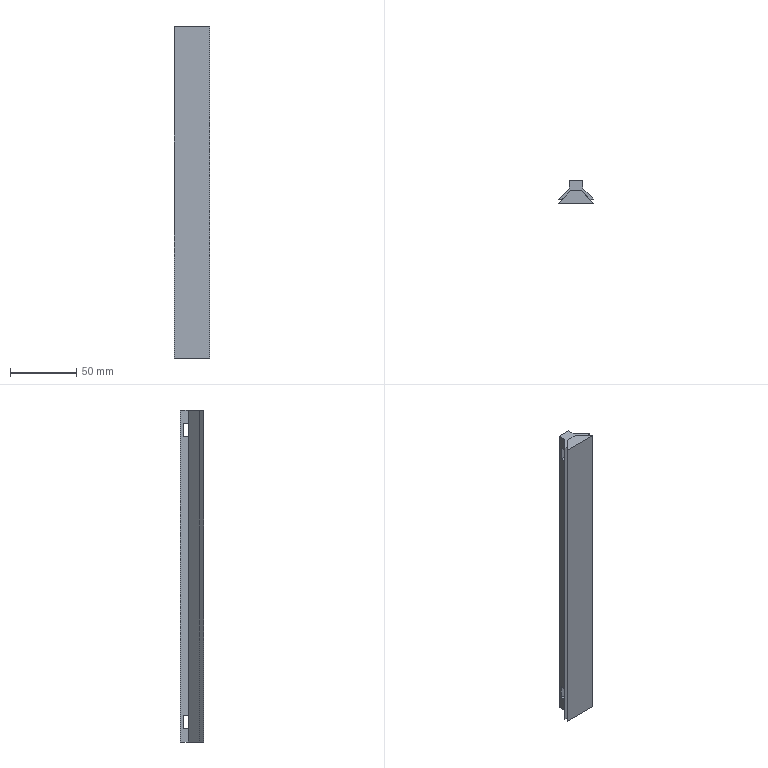Component | SolidWorks | Scraper-1 | 2 solids | 26 faces | box 26.97 x 17.45 x 250 mm | volume 70404 mm3 | plane 26
build123d program:
from build123d import *

# Parameters (mm, degrees)
BOSS_EXTRUDE1_DEPTH = 125
SKETCH3_W           = 250
SKETCH3_H           = 10
BOSS_EXTRUDE2_DEPTH = 6
SKETCH4_W           = 10
SKETCH4_H           = 4
CUT_EXTRUDE1_DEPTH  = 10
BOSS_EXTRUDE3_DEPTH = 250


with BuildPart() as part:
    # Sketch2 → Boss-Extrude1 (new, symmetric)
    with BuildSketch(Plane(origin=(0, 0, 0), x_dir=(0, 0, -1), z_dir=(1, 0, 0))):
        Polygon((-5, 0), (5, 0), (13.266, -8.266), (10.438, -8.266), (4.172, -2), (-4.172, -2), (-10.657, -8.485), (-13.485, -8.485), align=None)
    extrude(amount=BOSS_EXTRUDE1_DEPTH, both=True)

    # Sketch3 → Boss-Extrude2 (add)
    with BuildSketch(Plane(origin=(0, 0, 0), x_dir=(1, 0, 0), z_dir=(0, 1, 0))):
        Rectangle(SKETCH3_W, SKETCH3_H)
    extrude(amount=BOSS_EXTRUDE2_DEPTH)

    # Sketch4 → Cut-Extrude1 (cut)
    with BuildSketch(Plane.XY.offset(5)):
        with Locations((-110, 2)):
            Rectangle(SKETCH4_W, SKETCH4_H)
        with Locations((110, 2)):
            Rectangle(SKETCH4_W, SKETCH4_H)
    extrude(amount=-CUT_EXTRUDE1_DEPTH, mode=Mode.SUBTRACT)


with BuildPart() as body_2:
    # Sketch5 → Boss-Extrude3 (new body)
    with BuildSketch(Plane.ZY.offset(125)):
        Polygon((-4.13, -2.1), (-13.484, -11.453), (13.484, -11.453), (4.13, -2.1), align=None)
    extrude(amount=-BOSS_EXTRUDE3_DEPTH)


solid = Compound([part.part, body_2.part])

# Placed as in the assembly
solid = solid.moved(Location((440.482, -390.1, -8.037), (0, -90, 0)))
STEP:
#1=COLOUR_RGB('',0.7922,0.8196,0.9333);
#2=FILL_AREA_STYLE_COLOUR('',#1);
#3=FILL_AREA_STYLE('',(#2));
#4=SURFACE_STYLE_FILL_AREA(#3);
#5=SURFACE_SIDE_STYLE('',(#4));
#6=SURFACE_STYLE_USAGE(.BOTH.,#5);
#7=PRESENTATION_STYLE_ASSIGNMENT((#6));
#8=CARTESIAN_POINT('',(17.145,-15.358,-5.238));
#9=VERTEX_POINT('',#8);
#10=CARTESIAN_POINT('',(16.811,-15.692,-5.238));
#11=VERTEX_POINT('',#10);
#12=CARTESIAN_POINT('',(17.145,-15.358,-5.238));
#13=DIRECTION('',(-0.7071,-0.7071,-0.));
#14=VECTOR('',#13,39.37);
#15=LINE('',#12,#14);
#16=EDGE_CURVE('',#9,#11,#15,.T.);
#17=ORIENTED_EDGE('',*,*,#16,.T.);
#18=CARTESIAN_POINT('',(16.811,-15.692,4.605));
#19=VERTEX_POINT('',#18);
#20=CARTESIAN_POINT('',(16.811,-15.692,4.605));
#21=DIRECTION('',(0.,-0.,-1.));
#22=VECTOR('',#21,39.37);
#23=LINE('',#20,#22);
#24=EDGE_CURVE('',#19,#11,#23,.T.);
#25=ORIENTED_EDGE('',*,*,#24,.F.);
#26=CARTESIAN_POINT('',(17.145,-15.358,4.605));
#27=VERTEX_POINT('',#26);
#28=CARTESIAN_POINT('',(17.145,-15.358,4.605));
#29=DIRECTION('',(-0.7071,-0.7071,-0.));
#30=VECTOR('',#29,39.37);
#31=LINE('',#28,#30);
#32=EDGE_CURVE('',#27,#19,#31,.T.);
#33=ORIENTED_EDGE('',*,*,#32,.F.);
#34=CARTESIAN_POINT('',(17.145,-15.358,4.211));
#35=VERTEX_POINT('',#34);
#36=CARTESIAN_POINT('',(17.145,-15.358,4.605));
#37=DIRECTION('',(0.,-0.,-1.));
#38=VECTOR('',#37,39.37);
#39=LINE('',#36,#38);
#40=EDGE_CURVE('',#27,#35,#39,.T.);
#41=ORIENTED_EDGE('',*,*,#40,.T.);
#42=CARTESIAN_POINT('',(17.145,-15.358,3.817));
#43=VERTEX_POINT('',#42);
#44=CARTESIAN_POINT('',(17.145,-15.358,4.211));
#45=DIRECTION('',(-0.,0.,1.));
#46=VECTOR('',#45,39.37);
#47=LINE('',#44,#46);
#48=EDGE_CURVE('',#43,#35,#47,.T.);
#49=ORIENTED_EDGE('',*,*,#48,.F.);
#50=CARTESIAN_POINT('',(17.145,-15.358,-4.45));
#51=VERTEX_POINT('',#50);
#52=CARTESIAN_POINT('',(17.145,-15.358,4.605));
#53=DIRECTION('',(0.,-0.,-1.));
#54=VECTOR('',#53,39.37);
#55=LINE('',#52,#54);
#56=EDGE_CURVE('',#43,#51,#55,.T.);
#57=ORIENTED_EDGE('',*,*,#56,.T.);
#58=CARTESIAN_POINT('',(17.145,-15.358,-4.844));
#59=VERTEX_POINT('',#58);
#60=CARTESIAN_POINT('',(17.145,-15.358,-4.844));
#61=DIRECTION('',(-0.,0.,1.));
#62=VECTOR('',#61,39.37);
#63=LINE('',#60,#62);
#64=EDGE_CURVE('',#59,#51,#63,.T.);
#65=ORIENTED_EDGE('',*,*,#64,.F.);
#66=CARTESIAN_POINT('',(17.145,-15.358,4.605));
#67=DIRECTION('',(0.,-0.,-1.));
#68=VECTOR('',#67,39.37);
#69=LINE('',#66,#68);
#70=EDGE_CURVE('',#59,#9,#69,.T.);
#71=ORIENTED_EDGE('',*,*,#70,.T.);
#72=EDGE_LOOP('',(#17,#25,#33,#41,#49,#57,#65,#71));
#73=FACE_OUTER_BOUND('',#72,.T.);
#74=CARTESIAN_POINT('',(17.145,-15.358,4.605));
#75=DIRECTION('',(0.7071,-0.7071,0.));
#76=DIRECTION('',(0.7071,0.7071,0.));
#77=AXIS2_PLACEMENT_3D('',#74,#75,#76);
#78=PLANE('',#77);
#79=ADVANCED_FACE('',(#73),#78,.F.);
#80=CARTESIAN_POINT('',(16.922,-15.692,-5.238));
#81=VERTEX_POINT('',#80);
#82=CARTESIAN_POINT('',(16.922,-15.692,-5.238));
#83=DIRECTION('',(1.,0.,0.));
#84=VECTOR('',#83,39.37);
#85=LINE('',#82,#84);
#86=EDGE_CURVE('',#11,#81,#85,.T.);
#87=ORIENTED_EDGE('',*,*,#86,.T.);
#88=CARTESIAN_POINT('',(16.922,-15.692,4.605));
#89=VERTEX_POINT('',#88);
#90=CARTESIAN_POINT('',(16.922,-15.692,4.605));
#91=DIRECTION('',(0.,-0.,-1.));
#92=VECTOR('',#91,39.37);
#93=LINE('',#90,#92);
#94=EDGE_CURVE('',#89,#81,#93,.T.);
#95=ORIENTED_EDGE('',*,*,#94,.F.);
#96=CARTESIAN_POINT('',(16.922,-15.692,4.605));
#97=DIRECTION('',(1.,0.,0.));
#98=VECTOR('',#97,39.37);
#99=LINE('',#96,#98);
#100=EDGE_CURVE('',#19,#89,#99,.T.);
#101=ORIENTED_EDGE('',*,*,#100,.F.);
#102=ORIENTED_EDGE('',*,*,#24,.T.);
#103=EDGE_LOOP('',(#87,#95,#101,#102));
#104=FACE_OUTER_BOUND('',#103,.T.);
#105=CARTESIAN_POINT('',(16.922,-15.692,4.605));
#106=DIRECTION('',(-0.,1.,-0.));
#107=DIRECTION('',(-1.,-0.,-0.));
#108=AXIS2_PLACEMENT_3D('',#105,#106,#107);
#109=PLANE('',#108);
#110=ADVANCED_FACE('',(#104),#109,.F.);
#111=CARTESIAN_POINT('',(17.178,-15.437,-5.238));
#112=VERTEX_POINT('',#111);
#113=CARTESIAN_POINT('',(17.178,-15.437,-5.238));
#114=DIRECTION('',(0.7071,0.7071,0.));
#115=VECTOR('',#114,39.37);
#116=LINE('',#113,#115);
#117=EDGE_CURVE('',#81,#112,#116,.T.);
#118=ORIENTED_EDGE('',*,*,#117,.T.);
#119=CARTESIAN_POINT('',(17.178,-15.437,4.605));
#120=VERTEX_POINT('',#119);
#121=CARTESIAN_POINT('',(17.178,-15.437,4.605));
#122=DIRECTION('',(0.,-0.,-1.));
#123=VECTOR('',#122,39.37);
#124=LINE('',#121,#123);
#125=EDGE_CURVE('',#120,#112,#124,.T.);
#126=ORIENTED_EDGE('',*,*,#125,.F.);
#127=CARTESIAN_POINT('',(17.178,-15.437,4.605));
#128=DIRECTION('',(0.7071,0.7071,0.));
#129=VECTOR('',#128,39.37);
#130=LINE('',#127,#129);
#131=EDGE_CURVE('',#89,#120,#130,.T.);
#132=ORIENTED_EDGE('',*,*,#131,.F.);
#133=ORIENTED_EDGE('',*,*,#94,.T.);
#134=EDGE_LOOP('',(#118,#126,#132,#133));
#135=FACE_OUTER_BOUND('',#134,.T.);
#136=CARTESIAN_POINT('',(17.178,-15.437,4.605));
#137=DIRECTION('',(-0.7071,0.7071,-0.));
#138=DIRECTION('',(-0.7071,-0.7071,-0.));
#139=AXIS2_PLACEMENT_3D('',#136,#137,#138);
#140=PLANE('',#139);
#141=ADVANCED_FACE('',(#135),#140,.F.);
#142=CARTESIAN_POINT('',(17.506,-15.437,-5.238));
#143=VERTEX_POINT('',#142);
#144=CARTESIAN_POINT('',(17.178,-15.437,-5.238));
#145=DIRECTION('',(1.,0.,0.));
#146=VECTOR('',#145,39.37);
#147=LINE('',#144,#146);
#148=EDGE_CURVE('',#112,#143,#147,.T.);
#149=ORIENTED_EDGE('',*,*,#148,.T.);
#150=CARTESIAN_POINT('',(17.506,-15.437,4.605));
#151=VERTEX_POINT('',#150);
#152=CARTESIAN_POINT('',(17.506,-15.437,4.605));
#153=DIRECTION('',(0.,-0.,-1.));
#154=VECTOR('',#153,39.37);
#155=LINE('',#152,#154);
#156=EDGE_CURVE('',#151,#143,#155,.T.);
#157=ORIENTED_EDGE('',*,*,#156,.F.);
#158=CARTESIAN_POINT('',(17.178,-15.437,4.605));
#159=DIRECTION('',(1.,0.,0.));
#160=VECTOR('',#159,39.37);
#161=LINE('',#158,#160);
#162=EDGE_CURVE('',#120,#151,#161,.T.);
#163=ORIENTED_EDGE('',*,*,#162,.F.);
#164=ORIENTED_EDGE('',*,*,#125,.T.);
#165=EDGE_LOOP('',(#149,#157,#163,#164));
#166=FACE_OUTER_BOUND('',#165,.T.);
#167=CARTESIAN_POINT('',(17.178,-15.437,4.605));
#168=DIRECTION('',(-0.,1.,-0.));
#169=DIRECTION('',(-1.,-0.,-0.));
#170=AXIS2_PLACEMENT_3D('',#167,#168,#169);
#171=PLANE('',#170);
#172=ADVANCED_FACE('',(#166),#171,.F.);
#173=CARTESIAN_POINT('',(17.753,-15.684,-5.238));
#174=VERTEX_POINT('',#173);
#175=CARTESIAN_POINT('',(17.506,-15.437,-5.238));
#176=DIRECTION('',(0.7071,-0.7071,0.));
#177=VECTOR('',#176,39.37);
#178=LINE('',#175,#177);
#179=EDGE_CURVE('',#143,#174,#178,.T.);
#180=ORIENTED_EDGE('',*,*,#179,.T.);
#181=CARTESIAN_POINT('',(17.753,-15.684,4.605));
#182=VERTEX_POINT('',#181);
#183=CARTESIAN_POINT('',(17.753,-15.684,4.605));
#184=DIRECTION('',(0.,-0.,-1.));
#185=VECTOR('',#184,39.37);
#186=LINE('',#183,#185);
#187=EDGE_CURVE('',#182,#174,#186,.T.);
#188=ORIENTED_EDGE('',*,*,#187,.F.);
#189=CARTESIAN_POINT('',(17.506,-15.437,4.605));
#190=DIRECTION('',(0.7071,-0.7071,0.));
#191=VECTOR('',#190,39.37);
#192=LINE('',#189,#191);
#193=EDGE_CURVE('',#151,#182,#192,.T.);
#194=ORIENTED_EDGE('',*,*,#193,.F.);
#195=ORIENTED_EDGE('',*,*,#156,.T.);
#196=EDGE_LOOP('',(#180,#188,#194,#195));
#197=FACE_OUTER_BOUND('',#196,.T.);
#198=CARTESIAN_POINT('',(17.506,-15.437,4.605));
#199=DIRECTION('',(0.7071,0.7071,0.));
#200=DIRECTION('',(-0.7071,0.7071,-0.));
#201=AXIS2_PLACEMENT_3D('',#198,#199,#200);
#202=PLANE('',#201);
#203=ADVANCED_FACE('',(#197),#202,.F.);
#204=CARTESIAN_POINT('',(17.864,-15.684,-5.238));
#205=VERTEX_POINT('',#204);
#206=CARTESIAN_POINT('',(17.753,-15.684,-5.238));
#207=DIRECTION('',(1.,0.,0.));
#208=VECTOR('',#207,39.37);
#209=LINE('',#206,#208);
#210=EDGE_CURVE('',#174,#205,#209,.T.);
#211=ORIENTED_EDGE('',*,*,#210,.T.);
#212=CARTESIAN_POINT('',(17.864,-15.684,4.605));
#213=VERTEX_POINT('',#212);
#214=CARTESIAN_POINT('',(17.864,-15.684,4.605));
#215=DIRECTION('',(0.,-0.,-1.));
#216=VECTOR('',#215,39.37);
#217=LINE('',#214,#216);
#218=EDGE_CURVE('',#213,#205,#217,.T.);
#219=ORIENTED_EDGE('',*,*,#218,.F.);
#220=CARTESIAN_POINT('',(17.753,-15.684,4.605));
#221=DIRECTION('',(1.,0.,0.));
#222=VECTOR('',#221,39.37);
#223=LINE('',#220,#222);
#224=EDGE_CURVE('',#182,#213,#223,.T.);
#225=ORIENTED_EDGE('',*,*,#224,.F.);
#226=ORIENTED_EDGE('',*,*,#187,.T.);
#227=EDGE_LOOP('',(#211,#219,#225,#226));
#228=FACE_OUTER_BOUND('',#227,.T.);
#229=CARTESIAN_POINT('',(17.753,-15.684,4.605));
#230=DIRECTION('',(-0.,1.,-0.));
#231=DIRECTION('',(-1.,-0.,-0.));
#232=AXIS2_PLACEMENT_3D('',#229,#230,#231);
#233=PLANE('',#232);
#234=ADVANCED_FACE('',(#228),#233,.F.);
#235=CARTESIAN_POINT('',(17.539,-15.358,-5.238));
#236=VERTEX_POINT('',#235);
#237=CARTESIAN_POINT('',(17.539,-15.358,-5.238));
#238=DIRECTION('',(-0.7071,0.7071,-0.));
#239=VECTOR('',#238,39.37);
#240=LINE('',#237,#239);
#241=EDGE_CURVE('',#205,#236,#240,.T.);
#242=ORIENTED_EDGE('',*,*,#241,.T.);
#243=CARTESIAN_POINT('',(17.539,-15.358,-4.844));
#244=VERTEX_POINT('',#243);
#245=CARTESIAN_POINT('',(17.539,-15.358,4.605));
#246=DIRECTION('',(0.,-0.,-1.));
#247=VECTOR('',#246,39.37);
#248=LINE('',#245,#247);
#249=EDGE_CURVE('',#244,#236,#248,.T.);
#250=ORIENTED_EDGE('',*,*,#249,.F.);
#251=CARTESIAN_POINT('',(17.539,-15.358,-4.45));
#252=VERTEX_POINT('',#251);
#253=CARTESIAN_POINT('',(17.539,-15.358,-4.844));
#254=DIRECTION('',(-0.,0.,1.));
#255=VECTOR('',#254,39.37);
#256=LINE('',#253,#255);
#257=EDGE_CURVE('',#244,#252,#256,.T.);
#258=ORIENTED_EDGE('',*,*,#257,.T.);
#259=CARTESIAN_POINT('',(17.539,-15.358,3.817));
#260=VERTEX_POINT('',#259);
#261=CARTESIAN_POINT('',(17.539,-15.358,4.605));
#262=DIRECTION('',(0.,-0.,-1.));
#263=VECTOR('',#262,39.37);
#264=LINE('',#261,#263);
#265=EDGE_CURVE('',#260,#252,#264,.T.);
#266=ORIENTED_EDGE('',*,*,#265,.F.);
#267=CARTESIAN_POINT('',(17.539,-15.358,4.211));
#268=VERTEX_POINT('',#267);
#269=CARTESIAN_POINT('',(17.539,-15.358,4.211));
#270=DIRECTION('',(-0.,0.,1.));
#271=VECTOR('',#270,39.37);
#272=LINE('',#269,#271);
#273=EDGE_CURVE('',#260,#268,#272,.T.);
#274=ORIENTED_EDGE('',*,*,#273,.T.);
#275=CARTESIAN_POINT('',(17.539,-15.358,4.605));
#276=VERTEX_POINT('',#275);
#277=CARTESIAN_POINT('',(17.539,-15.358,4.605));
#278=DIRECTION('',(0.,-0.,-1.));
#279=VECTOR('',#278,39.37);
#280=LINE('',#277,#279);
#281=EDGE_CURVE('',#276,#268,#280,.T.);
#282=ORIENTED_EDGE('',*,*,#281,.F.);
#283=CARTESIAN_POINT('',(17.539,-15.358,4.605));
#284=DIRECTION('',(-0.7071,0.7071,-0.));
#285=VECTOR('',#284,39.37);
#286=LINE('',#283,#285);
#287=EDGE_CURVE('',#213,#276,#286,.T.);
#288=ORIENTED_EDGE('',*,*,#287,.F.);
#289=ORIENTED_EDGE('',*,*,#218,.T.);
#290=EDGE_LOOP('',(#242,#250,#258,#266,#274,#282,#288,#289));
#291=FACE_OUTER_BOUND('',#290,.T.);
#292=CARTESIAN_POINT('',(17.539,-15.358,4.605));
#293=DIRECTION('',(-0.7071,-0.7071,-0.));
#294=DIRECTION('',(0.7071,-0.7071,0.));
#295=AXIS2_PLACEMENT_3D('',#292,#293,#294);
#296=PLANE('',#295);
#297=ADVANCED_FACE('',(#291),#296,.F.);
#298=ORIENTED_EDGE('',*,*,#32,.T.);
#299=ORIENTED_EDGE('',*,*,#100,.T.);
#300=ORIENTED_EDGE('',*,*,#131,.T.);
#301=ORIENTED_EDGE('',*,*,#162,.T.);
#302=ORIENTED_EDGE('',*,*,#193,.T.);
#303=ORIENTED_EDGE('',*,*,#224,.T.);
#304=ORIENTED_EDGE('',*,*,#287,.T.);
#305=CARTESIAN_POINT('',(17.539,-15.122,4.605));
#306=VERTEX_POINT('',#305);
#307=CARTESIAN_POINT('',(17.539,-15.122,4.605));
#308=DIRECTION('',(0.,-1.,0.));
#309=VECTOR('',#308,39.37);
#310=LINE('',#307,#309);
#311=EDGE_CURVE('',#306,#276,#310,.T.);
#312=ORIENTED_EDGE('',*,*,#311,.F.);
#313=CARTESIAN_POINT('',(17.145,-15.122,4.605));
#314=VERTEX_POINT('',#313);
#315=CARTESIAN_POINT('',(17.145,-15.122,4.605));
#316=DIRECTION('',(1.,0.,0.));
#317=VECTOR('',#316,39.37);
#318=LINE('',#315,#317);
#319=EDGE_CURVE('',#314,#306,#318,.T.);
#320=ORIENTED_EDGE('',*,*,#319,.F.);
#321=CARTESIAN_POINT('',(17.145,-15.122,4.605));
#322=DIRECTION('',(0.,-1.,0.));
#323=VECTOR('',#322,39.37);
#324=LINE('',#321,#323);
#325=EDGE_CURVE('',#314,#27,#324,.T.);
#326=ORIENTED_EDGE('',*,*,#325,.T.);
#327=EDGE_LOOP('',(#298,#299,#300,#301,#302,#303,#304,#312,#320,#326));
#328=FACE_OUTER_BOUND('',#327,.T.);
#329=CARTESIAN_POINT('',(17.342,-15.358,4.605));
#330=DIRECTION('',(-0.,0.,1.));
#331=DIRECTION('',(1.,0.,0.));
#332=AXIS2_PLACEMENT_3D('',#329,#330,#331);
#333=PLANE('',#332);
#334=ADVANCED_FACE('',(#328),#333,.T.);
#335=ORIENTED_EDGE('',*,*,#16,.F.);
#336=CARTESIAN_POINT('',(17.145,-15.122,-5.238));
#337=VERTEX_POINT('',#336);
#338=CARTESIAN_POINT('',(17.145,-15.122,-5.238));
#339=DIRECTION('',(0.,-1.,0.));
#340=VECTOR('',#339,39.37);
#341=LINE('',#338,#340);
#342=EDGE_CURVE('',#337,#9,#341,.T.);
#343=ORIENTED_EDGE('',*,*,#342,.F.);
#344=CARTESIAN_POINT('',(17.539,-15.122,-5.238));
#345=VERTEX_POINT('',#344);
#346=CARTESIAN_POINT('',(17.145,-15.122,-5.238));
#347=DIRECTION('',(-1.,-0.,-0.));
#348=VECTOR('',#347,39.37);
#349=LINE('',#346,#348);
#350=EDGE_CURVE('',#345,#337,#349,.T.);
#351=ORIENTED_EDGE('',*,*,#350,.F.);
#352=CARTESIAN_POINT('',(17.539,-15.122,-5.238));
#353=DIRECTION('',(0.,-1.,0.));
#354=VECTOR('',#353,39.37);
#355=LINE('',#352,#354);
#356=EDGE_CURVE('',#345,#236,#355,.T.);
#357=ORIENTED_EDGE('',*,*,#356,.T.);
#358=ORIENTED_EDGE('',*,*,#241,.F.);
#359=ORIENTED_EDGE('',*,*,#210,.F.);
#360=ORIENTED_EDGE('',*,*,#179,.F.);
#361=ORIENTED_EDGE('',*,*,#148,.F.);
#362=ORIENTED_EDGE('',*,*,#117,.F.);
#363=ORIENTED_EDGE('',*,*,#86,.F.);
#364=EDGE_LOOP('',(#335,#343,#351,#357,#358,#359,#360,#361,#362,#363));
#365=FACE_OUTER_BOUND('',#364,.T.);
#366=CARTESIAN_POINT('',(17.342,-15.358,-5.238));
#367=DIRECTION('',(-0.,0.,1.));
#368=DIRECTION('',(1.,0.,0.));
#369=AXIS2_PLACEMENT_3D('',#366,#367,#368);
#370=PLANE('',#369);
#371=ADVANCED_FACE('',(#365),#370,.F.);
#372=ORIENTED_EDGE('',*,*,#281,.T.);
#373=CARTESIAN_POINT('',(17.539,-15.201,4.211));
#374=VERTEX_POINT('',#373);
#375=CARTESIAN_POINT('',(17.539,-15.201,4.211));
#376=DIRECTION('',(-0.,1.,-0.));
#377=VECTOR('',#376,39.37);
#378=LINE('',#375,#377);
#379=EDGE_CURVE('',#268,#374,#378,.T.);
#380=ORIENTED_EDGE('',*,*,#379,.T.);
#381=CARTESIAN_POINT('',(17.539,-15.201,3.817));
#382=VERTEX_POINT('',#381);
#383=CARTESIAN_POINT('',(17.539,-15.201,3.817));
#384=DIRECTION('',(0.,-0.,-1.));
#385=VECTOR('',#384,39.37);
#386=LINE('',#383,#385);
#387=EDGE_CURVE('',#374,#382,#386,.T.);
#388=ORIENTED_EDGE('',*,*,#387,.T.);
#389=CARTESIAN_POINT('',(17.539,-15.358,3.817));
#390=DIRECTION('',(0.,-1.,0.));
#391=VECTOR('',#390,39.37);
#392=LINE('',#389,#391);
#393=EDGE_CURVE('',#382,#260,#392,.T.);
#394=ORIENTED_EDGE('',*,*,#393,.T.);
#395=ORIENTED_EDGE('',*,*,#265,.T.);
#396=CARTESIAN_POINT('',(17.539,-15.201,-4.45));
#397=VERTEX_POINT('',#396);
#398=CARTESIAN_POINT('',(17.539,-15.358,-4.45));
#399=DIRECTION('',(-0.,1.,-0.));
#400=VECTOR('',#399,39.37);
#401=LINE('',#398,#400);
#402=EDGE_CURVE('',#252,#397,#401,.T.);
#403=ORIENTED_EDGE('',*,*,#402,.T.);
#404=CARTESIAN_POINT('',(17.539,-15.201,-4.844));
#405=VERTEX_POINT('',#404);
#406=CARTESIAN_POINT('',(17.539,-15.201,-4.45));
#407=DIRECTION('',(0.,-0.,-1.));
#408=VECTOR('',#407,39.37);
#409=LINE('',#406,#408);
#410=EDGE_CURVE('',#397,#405,#409,.T.);
#411=ORIENTED_EDGE('',*,*,#410,.T.);
#412=CARTESIAN_POINT('',(17.539,-15.201,-4.844));
#413=DIRECTION('',(0.,-1.,0.));
#414=VECTOR('',#413,39.37);
#415=LINE('',#412,#414);
#416=EDGE_CURVE('',#405,#244,#415,.T.);
#417=ORIENTED_EDGE('',*,*,#416,.T.);
#418=ORIENTED_EDGE('',*,*,#249,.T.);
#419=ORIENTED_EDGE('',*,*,#356,.F.);
#420=CARTESIAN_POINT('',(17.539,-15.122,-5.238));
#421=DIRECTION('',(0.,-0.,-1.));
#422=VECTOR('',#421,39.37);
#423=LINE('',#420,#422);
#424=EDGE_CURVE('',#306,#345,#423,.T.);
#425=ORIENTED_EDGE('',*,*,#424,.F.);
#426=ORIENTED_EDGE('',*,*,#311,.T.);
#427=EDGE_LOOP('',(#372,#380,#388,#394,#395,#403,#411,#417,#418,#419,#425,#426));
#428=FACE_OUTER_BOUND('',#427,.T.);
#429=CARTESIAN_POINT('',(17.539,-15.122,-5.238));
#430=DIRECTION('',(-1.,-0.,-0.));
#431=DIRECTION('',(0.,-1.,0.));
#432=AXIS2_PLACEMENT_3D('',#429,#430,#431);
#433=PLANE('',#432);
#434=ADVANCED_FACE('',(#428),#433,.F.);
#435=CARTESIAN_POINT('',(17.145,-15.201,4.211));
#436=VERTEX_POINT('',#435);
#437=CARTESIAN_POINT('',(17.145,-15.201,3.817));
#438=VERTEX_POINT('',#437);
#439=CARTESIAN_POINT('',(17.145,-15.201,3.817));
#440=DIRECTION('',(0.,-0.,-1.));
#441=VECTOR('',#440,39.37);
#442=LINE('',#439,#441);
#443=EDGE_CURVE('',#436,#438,#442,.T.);
#444=ORIENTED_EDGE('',*,*,#443,.F.);
#445=CARTESIAN_POINT('',(17.145,-15.201,4.211));
#446=DIRECTION('',(-0.,1.,-0.));
#447=VECTOR('',#446,39.37);
#448=LINE('',#445,#447);
#449=EDGE_CURVE('',#35,#436,#448,.T.);
#450=ORIENTED_EDGE('',*,*,#449,.F.);
#451=ORIENTED_EDGE('',*,*,#40,.F.);
#452=ORIENTED_EDGE('',*,*,#325,.F.);
#453=CARTESIAN_POINT('',(17.145,-15.122,-5.238));
#454=DIRECTION('',(-0.,0.,1.));
#455=VECTOR('',#454,39.37);
#456=LINE('',#453,#455);
#457=EDGE_CURVE('',#337,#314,#456,.T.);
#458=ORIENTED_EDGE('',*,*,#457,.F.);
#459=ORIENTED_EDGE('',*,*,#342,.T.);
#460=ORIENTED_EDGE('',*,*,#70,.F.);
#461=CARTESIAN_POINT('',(17.145,-15.201,-4.844));
#462=VERTEX_POINT('',#461);
#463=CARTESIAN_POINT('',(17.145,-15.201,-4.844));
#464=DIRECTION('',(0.,-1.,0.));
#465=VECTOR('',#464,39.37);
#466=LINE('',#463,#465);
#467=EDGE_CURVE('',#462,#59,#466,.T.);
#468=ORIENTED_EDGE('',*,*,#467,.F.);
#469=CARTESIAN_POINT('',(17.145,-15.201,-4.45));
#470=VERTEX_POINT('',#469);
#471=CARTESIAN_POINT('',(17.145,-15.201,-4.45));
#472=DIRECTION('',(0.,-0.,-1.));
#473=VECTOR('',#472,39.37);
#474=LINE('',#471,#473);
#475=EDGE_CURVE('',#470,#462,#474,.T.);
#476=ORIENTED_EDGE('',*,*,#475,.F.);
#477=CARTESIAN_POINT('',(17.145,-15.358,-4.45));
#478=DIRECTION('',(-0.,1.,-0.));
#479=VECTOR('',#478,39.37);
#480=LINE('',#477,#479);
#481=EDGE_CURVE('',#51,#470,#480,.T.);
#482=ORIENTED_EDGE('',*,*,#481,.F.);
#483=ORIENTED_EDGE('',*,*,#56,.F.);
#484=CARTESIAN_POINT('',(17.145,-15.358,3.817));
#485=DIRECTION('',(0.,-1.,0.));
#486=VECTOR('',#485,39.37);
#487=LINE('',#484,#486);
#488=EDGE_CURVE('',#438,#43,#487,.T.);
#489=ORIENTED_EDGE('',*,*,#488,.F.);
#490=EDGE_LOOP('',(#444,#450,#451,#452,#458,#459,#460,#468,#476,#482,#483,#489));
#491=FACE_OUTER_BOUND('',#490,.T.);
#492=CARTESIAN_POINT('',(17.145,-15.122,-5.238));
#493=DIRECTION('',(1.,0.,0.));
#494=DIRECTION('',(-0.,1.,-0.));
#495=AXIS2_PLACEMENT_3D('',#492,#493,#494);
#496=PLANE('',#495);
#497=ADVANCED_FACE('',(#491),#496,.F.);
#498=ORIENTED_EDGE('',*,*,#319,.T.);
#499=ORIENTED_EDGE('',*,*,#424,.T.);
#500=ORIENTED_EDGE('',*,*,#350,.T.);
#501=ORIENTED_EDGE('',*,*,#457,.T.);
#502=EDGE_LOOP('',(#498,#499,#500,#501));
#503=FACE_OUTER_BOUND('',#502,.T.);
#504=CARTESIAN_POINT('',(17.342,-15.122,-0.3164));
#505=DIRECTION('',(0.,-1.,0.));
#506=DIRECTION('',(1.,0.,0.));
#507=AXIS2_PLACEMENT_3D('',#504,#505,#506);
#508=PLANE('',#507);
#509=ADVANCED_FACE('',(#503),#508,.F.);
#510=ORIENTED_EDGE('',*,*,#64,.T.);
#511=CARTESIAN_POINT('',(17.539,-15.358,-4.45));
#512=DIRECTION('',(-1.,-0.,-0.));
#513=VECTOR('',#512,39.37);
#514=LINE('',#511,#513);
#515=EDGE_CURVE('',#252,#51,#514,.T.);
#516=ORIENTED_EDGE('',*,*,#515,.F.);
#517=ORIENTED_EDGE('',*,*,#257,.F.);
#518=CARTESIAN_POINT('',(17.539,-15.358,-4.844));
#519=DIRECTION('',(-1.,-0.,-0.));
#520=VECTOR('',#519,39.37);
#521=LINE('',#518,#520);
#522=EDGE_CURVE('',#244,#59,#521,.T.);
#523=ORIENTED_EDGE('',*,*,#522,.T.);
#524=EDGE_LOOP('',(#510,#516,#517,#523));
#525=FACE_OUTER_BOUND('',#524,.T.);
#526=CARTESIAN_POINT('',(17.539,-15.358,-4.844));
#527=DIRECTION('',(0.,-1.,0.));
#528=DIRECTION('',(-0.,0.,1.));
#529=AXIS2_PLACEMENT_3D('',#526,#527,#528);
#530=PLANE('',#529);
#531=ADVANCED_FACE('',(#525),#530,.F.);
#532=ORIENTED_EDGE('',*,*,#467,.T.);
#533=ORIENTED_EDGE('',*,*,#522,.F.);
#534=ORIENTED_EDGE('',*,*,#416,.F.);
#535=CARTESIAN_POINT('',(17.539,-15.201,-4.844));
#536=DIRECTION('',(-1.,-0.,-0.));
#537=VECTOR('',#536,39.37);
#538=LINE('',#535,#537);
#539=EDGE_CURVE('',#405,#462,#538,.T.);
#540=ORIENTED_EDGE('',*,*,#539,.T.);
#541=EDGE_LOOP('',(#532,#533,#534,#540));
#542=FACE_OUTER_BOUND('',#541,.T.);
#543=CARTESIAN_POINT('',(17.539,-15.201,-4.844));
#544=DIRECTION('',(0.,-0.,-1.));
#545=DIRECTION('',(-1.,-0.,-0.));
#546=AXIS2_PLACEMENT_3D('',#543,#544,#545);
#547=PLANE('',#546);
#548=ADVANCED_FACE('',(#542),#547,.F.);
#549=ORIENTED_EDGE('',*,*,#475,.T.);
#550=ORIENTED_EDGE('',*,*,#539,.F.);
#551=ORIENTED_EDGE('',*,*,#410,.F.);
#552=CARTESIAN_POINT('',(17.539,-15.201,-4.45));
#553=DIRECTION('',(-1.,-0.,-0.));
#554=VECTOR('',#553,39.37);
#555=LINE('',#552,#554);
#556=EDGE_CURVE('',#397,#470,#555,.T.);
#557=ORIENTED_EDGE('',*,*,#556,.T.);
#558=EDGE_LOOP('',(#549,#550,#551,#557));
#559=FACE_OUTER_BOUND('',#558,.T.);
#560=CARTESIAN_POINT('',(17.539,-15.201,-4.45));
#561=DIRECTION('',(-0.,1.,-0.));
#562=DIRECTION('',(-1.,-0.,-0.));
#563=AXIS2_PLACEMENT_3D('',#560,#561,#562);
#564=PLANE('',#563);
#565=ADVANCED_FACE('',(#559),#564,.F.);
#566=ORIENTED_EDGE('',*,*,#481,.T.);
#567=ORIENTED_EDGE('',*,*,#556,.F.);
#568=ORIENTED_EDGE('',*,*,#402,.F.);
#569=ORIENTED_EDGE('',*,*,#515,.T.);
#570=EDGE_LOOP('',(#566,#567,#568,#569));
#571=FACE_OUTER_BOUND('',#570,.T.);
#572=CARTESIAN_POINT('',(17.539,-15.358,-4.45));
#573=DIRECTION('',(-0.,0.,1.));
#574=DIRECTION('',(1.,0.,0.));
#575=AXIS2_PLACEMENT_3D('',#572,#573,#574);
#576=PLANE('',#575);
#577=ADVANCED_FACE('',(#571),#576,.F.);
#578=ORIENTED_EDGE('',*,*,#449,.T.);
#579=CARTESIAN_POINT('',(17.539,-15.201,4.211));
#580=DIRECTION('',(-1.,-0.,-0.));
#581=VECTOR('',#580,39.37);
#582=LINE('',#579,#581);
#583=EDGE_CURVE('',#374,#436,#582,.T.);
#584=ORIENTED_EDGE('',*,*,#583,.F.);
#585=ORIENTED_EDGE('',*,*,#379,.F.);
#586=CARTESIAN_POINT('',(17.539,-15.358,4.211));
#587=DIRECTION('',(-1.,-0.,-0.));
#588=VECTOR('',#587,39.37);
#589=LINE('',#586,#588);
#590=EDGE_CURVE('',#268,#35,#589,.T.);
#591=ORIENTED_EDGE('',*,*,#590,.T.);
#592=EDGE_LOOP('',(#578,#584,#585,#591));
#593=FACE_OUTER_BOUND('',#592,.T.);
#594=CARTESIAN_POINT('',(17.539,-15.201,4.211));
#595=DIRECTION('',(-0.,0.,1.));
#596=DIRECTION('',(1.,0.,0.));
#597=AXIS2_PLACEMENT_3D('',#594,#595,#596);
#598=PLANE('',#597);
#599=ADVANCED_FACE('',(#593),#598,.F.);
#600=ORIENTED_EDGE('',*,*,#48,.T.);
#601=ORIENTED_EDGE('',*,*,#590,.F.);
#602=ORIENTED_EDGE('',*,*,#273,.F.);
#603=CARTESIAN_POINT('',(17.539,-15.358,3.817));
#604=DIRECTION('',(-1.,-0.,-0.));
#605=VECTOR('',#604,39.37);
#606=LINE('',#603,#605);
#607=EDGE_CURVE('',#260,#43,#606,.T.);
#608=ORIENTED_EDGE('',*,*,#607,.T.);
#609=EDGE_LOOP('',(#600,#601,#602,#608));
#610=FACE_OUTER_BOUND('',#609,.T.);
#611=CARTESIAN_POINT('',(17.539,-15.358,4.211));
#612=DIRECTION('',(0.,-1.,0.));
#613=DIRECTION('',(-0.,0.,1.));
#614=AXIS2_PLACEMENT_3D('',#611,#612,#613);
#615=PLANE('',#614);
#616=ADVANCED_FACE('',(#610),#615,.F.);
#617=ORIENTED_EDGE('',*,*,#488,.T.);
#618=ORIENTED_EDGE('',*,*,#607,.F.);
#619=ORIENTED_EDGE('',*,*,#393,.F.);
#620=CARTESIAN_POINT('',(17.539,-15.201,3.817));
#621=DIRECTION('',(-1.,-0.,-0.));
#622=VECTOR('',#621,39.37);
#623=LINE('',#620,#622);
#624=EDGE_CURVE('',#382,#438,#623,.T.);
#625=ORIENTED_EDGE('',*,*,#624,.T.);
#626=EDGE_LOOP('',(#617,#618,#619,#625));
#627=FACE_OUTER_BOUND('',#626,.T.);
#628=CARTESIAN_POINT('',(17.539,-15.358,3.817));
#629=DIRECTION('',(0.,-0.,-1.));
#630=DIRECTION('',(-1.,-0.,-0.));
#631=AXIS2_PLACEMENT_3D('',#628,#629,#630);
#632=PLANE('',#631);
#633=ADVANCED_FACE('',(#627),#632,.F.);
#634=ORIENTED_EDGE('',*,*,#443,.T.);
#635=ORIENTED_EDGE('',*,*,#624,.F.);
#636=ORIENTED_EDGE('',*,*,#387,.F.);
#637=ORIENTED_EDGE('',*,*,#583,.T.);
#638=EDGE_LOOP('',(#634,#635,#636,#637));
#639=FACE_OUTER_BOUND('',#638,.T.);
#640=CARTESIAN_POINT('',(17.539,-15.201,3.817));
#641=DIRECTION('',(-0.,1.,-0.));
#642=DIRECTION('',(-1.,-0.,-0.));
#643=AXIS2_PLACEMENT_3D('',#640,#641,#642);
#644=PLANE('',#643);
#645=ADVANCED_FACE('',(#639),#644,.F.);
#646=CLOSED_SHELL('',(#79,#110,#141,#172,#203,#234,#297,#334,#371,#434,#497,#509,#531,#548,#565,#577,#599,#616,#633,#645));
#647=MANIFOLD_SOLID_BREP('',#646);
#648=STYLED_ITEM('',(#7),#647);
#649=(LENGTH_UNIT()NAMED_UNIT(*)SI_UNIT($,.METRE.));
#650=LENGTH_MEASURE_WITH_UNIT(LENGTH_MEASURE(0.0254),#649);
#651=DIMENSIONAL_EXPONENTS(1.,0.,0.,0.,0.,0.,0.);
#652=(CONVERSION_BASED_UNIT('',#650)LENGTH_UNIT()NAMED_UNIT(#651));
#653=UNCERTAINTY_MEASURE_WITH_UNIT(LENGTH_MEASURE(0.00001),#652,'','');
#654=(NAMED_UNIT(*)PLANE_ANGLE_UNIT()SI_UNIT($,.RADIAN.));
#655=(NAMED_UNIT(*)SI_UNIT($,.STERADIAN.)SOLID_ANGLE_UNIT());
#656=(GEOMETRIC_REPRESENTATION_CONTEXT(3)GLOBAL_UNCERTAINTY_ASSIGNED_CONTEXT((#653))GLOBAL_UNIT_ASSIGNED_CONTEXT((#652,#654,#655))REPRESENTATION_CONTEXT('',''));
#657=MECHANICAL_DESIGN_GEOMETRIC_PRESENTATION_REPRESENTATION('',(#648),#656);
#658=PRESENTATION_LAYER_ASSIGNMENT('','',(#648));
#659=COLOUR_RGB('',0.7922,0.8196,0.9333);
#660=FILL_AREA_STYLE_COLOUR('',#659);
#661=FILL_AREA_STYLE('',(#660));
#662=SURFACE_STYLE_FILL_AREA(#661);
#663=SURFACE_SIDE_STYLE('',(#662));
#664=SURFACE_STYLE_USAGE(.BOTH.,#663);
#665=PRESENTATION_STYLE_ASSIGNMENT((#664));
#666=CARTESIAN_POINT('',(17.179,-15.441,4.605));
#667=VERTEX_POINT('',#666);
#668=CARTESIAN_POINT('',(17.504,-15.441,4.605));
#669=VERTEX_POINT('',#668);
#670=CARTESIAN_POINT('',(17.179,-15.441,4.605));
#671=DIRECTION('',(1.,0.,0.));
#672=VECTOR('',#671,39.37);
#673=LINE('',#670,#672);
#674=EDGE_CURVE('',#667,#669,#673,.T.);
#675=ORIENTED_EDGE('',*,*,#674,.F.);
#676=CARTESIAN_POINT('',(16.811,-15.809,4.605));
#677=VERTEX_POINT('',#676);
#678=CARTESIAN_POINT('',(16.811,-15.809,4.605));
#679=DIRECTION('',(0.7071,0.7071,0.));
#680=VECTOR('',#679,39.37);
#681=LINE('',#678,#680);
#682=EDGE_CURVE('',#677,#667,#681,.T.);
#683=ORIENTED_EDGE('',*,*,#682,.F.);
#684=CARTESIAN_POINT('',(17.873,-15.809,4.605));
#685=VERTEX_POINT('',#684);
#686=CARTESIAN_POINT('',(17.873,-15.809,4.605));
#687=DIRECTION('',(-1.,-0.,-0.));
#688=VECTOR('',#687,39.37);
#689=LINE('',#686,#688);
#690=EDGE_CURVE('',#685,#677,#689,.T.);
#691=ORIENTED_EDGE('',*,*,#690,.F.);
#692=CARTESIAN_POINT('',(17.504,-15.441,4.605));
#693=DIRECTION('',(0.7071,-0.7071,0.));
#694=VECTOR('',#693,39.37);
#695=LINE('',#692,#694);
#696=EDGE_CURVE('',#669,#685,#695,.T.);
#697=ORIENTED_EDGE('',*,*,#696,.F.);
#698=EDGE_LOOP('',(#675,#683,#691,#697));
#699=FACE_OUTER_BOUND('',#698,.T.);
#700=CARTESIAN_POINT('',(17.342,-15.358,4.605));
#701=DIRECTION('',(-0.,0.,1.));
#702=DIRECTION('',(1.,0.,0.));
#703=AXIS2_PLACEMENT_3D('',#700,#701,#702);
#704=PLANE('',#703);
#705=ADVANCED_FACE('',(#699),#704,.T.);
#706=CARTESIAN_POINT('',(17.179,-15.441,-5.238));
#707=VERTEX_POINT('',#706);
#708=CARTESIAN_POINT('',(17.504,-15.441,-5.238));
#709=VERTEX_POINT('',#708);
#710=CARTESIAN_POINT('',(17.179,-15.441,-5.238));
#711=DIRECTION('',(1.,0.,0.));
#712=VECTOR('',#711,39.37);
#713=LINE('',#710,#712);
#714=EDGE_CURVE('',#707,#709,#713,.T.);
#715=ORIENTED_EDGE('',*,*,#714,.T.);
#716=CARTESIAN_POINT('',(17.873,-15.809,-5.238));
#717=VERTEX_POINT('',#716);
#718=CARTESIAN_POINT('',(17.504,-15.441,-5.238));
#719=DIRECTION('',(0.7071,-0.7071,0.));
#720=VECTOR('',#719,39.37);
#721=LINE('',#718,#720);
#722=EDGE_CURVE('',#709,#717,#721,.T.);
#723=ORIENTED_EDGE('',*,*,#722,.T.);
#724=CARTESIAN_POINT('',(16.811,-15.809,-5.238));
#725=VERTEX_POINT('',#724);
#726=CARTESIAN_POINT('',(17.873,-15.809,-5.238));
#727=DIRECTION('',(-1.,-0.,-0.));
#728=VECTOR('',#727,39.37);
#729=LINE('',#726,#728);
#730=EDGE_CURVE('',#717,#725,#729,.T.);
#731=ORIENTED_EDGE('',*,*,#730,.T.);
#732=CARTESIAN_POINT('',(16.811,-15.809,-5.238));
#733=DIRECTION('',(0.7071,0.7071,0.));
#734=VECTOR('',#733,39.37);
#735=LINE('',#732,#734);
#736=EDGE_CURVE('',#725,#707,#735,.T.);
#737=ORIENTED_EDGE('',*,*,#736,.T.);
#738=EDGE_LOOP('',(#715,#723,#731,#737));
#739=FACE_OUTER_BOUND('',#738,.T.);
#740=CARTESIAN_POINT('',(17.342,-15.358,-5.238));
#741=DIRECTION('',(-0.,0.,1.));
#742=DIRECTION('',(1.,0.,0.));
#743=AXIS2_PLACEMENT_3D('',#740,#741,#742);
#744=PLANE('',#743);
#745=ADVANCED_FACE('',(#739),#744,.F.);
#746=CARTESIAN_POINT('',(17.504,-15.441,5.729));
#747=DIRECTION('',(0.,-0.,-1.));
#748=VECTOR('',#747,39.37);
#749=LINE('',#746,#748);
#750=EDGE_CURVE('',#669,#709,#749,.T.);
#751=ORIENTED_EDGE('',*,*,#750,.F.);
#752=ORIENTED_EDGE('',*,*,#696,.T.);
#753=CARTESIAN_POINT('',(17.873,-15.809,5.729));
#754=DIRECTION('',(0.,-0.,-1.));
#755=VECTOR('',#754,39.37);
#756=LINE('',#753,#755);
#757=EDGE_CURVE('',#685,#717,#756,.T.);
#758=ORIENTED_EDGE('',*,*,#757,.T.);
#759=ORIENTED_EDGE('',*,*,#722,.F.);
#760=EDGE_LOOP('',(#751,#752,#758,#759));
#761=FACE_OUTER_BOUND('',#760,.T.);
#762=CARTESIAN_POINT('',(17.504,-15.441,5.729));
#763=DIRECTION('',(0.7071,0.7071,0.));
#764=DIRECTION('',(-0.7071,0.7071,-0.));
#765=AXIS2_PLACEMENT_3D('',#762,#763,#764);
#766=PLANE('',#765);
#767=ADVANCED_FACE('',(#761),#766,.T.);
#768=ORIENTED_EDGE('',*,*,#757,.F.);
#769=ORIENTED_EDGE('',*,*,#690,.T.);
#770=CARTESIAN_POINT('',(16.811,-15.809,5.729));
#771=DIRECTION('',(0.,-0.,-1.));
#772=VECTOR('',#771,39.37);
#773=LINE('',#770,#772);
#774=EDGE_CURVE('',#677,#725,#773,.T.);
#775=ORIENTED_EDGE('',*,*,#774,.T.);
#776=ORIENTED_EDGE('',*,*,#730,.F.);
#777=EDGE_LOOP('',(#768,#769,#775,#776));
#778=FACE_OUTER_BOUND('',#777,.T.);
#779=CARTESIAN_POINT('',(17.873,-15.809,5.729));
#780=DIRECTION('',(0.,-1.,0.));
#781=DIRECTION('',(1.,0.,0.));
#782=AXIS2_PLACEMENT_3D('',#779,#780,#781);
#783=PLANE('',#782);
#784=ADVANCED_FACE('',(#778),#783,.T.);
#785=ORIENTED_EDGE('',*,*,#774,.F.);
#786=ORIENTED_EDGE('',*,*,#682,.T.);
#787=CARTESIAN_POINT('',(17.179,-15.441,5.729));
#788=DIRECTION('',(0.,-0.,-1.));
#789=VECTOR('',#788,39.37);
#790=LINE('',#787,#789);
#791=EDGE_CURVE('',#667,#707,#790,.T.);
#792=ORIENTED_EDGE('',*,*,#791,.T.);
#793=ORIENTED_EDGE('',*,*,#736,.F.);
#794=EDGE_LOOP('',(#785,#786,#792,#793));
#795=FACE_OUTER_BOUND('',#794,.T.);
#796=CARTESIAN_POINT('',(16.811,-15.809,5.729));
#797=DIRECTION('',(-0.7071,0.7071,-0.));
#798=DIRECTION('',(-0.7071,-0.7071,-0.));
#799=AXIS2_PLACEMENT_3D('',#796,#797,#798);
#800=PLANE('',#799);
#801=ADVANCED_FACE('',(#795),#800,.T.);
#802=ORIENTED_EDGE('',*,*,#791,.F.);
#803=ORIENTED_EDGE('',*,*,#674,.T.);
#804=ORIENTED_EDGE('',*,*,#750,.T.);
#805=ORIENTED_EDGE('',*,*,#714,.F.);
#806=EDGE_LOOP('',(#802,#803,#804,#805));
#807=FACE_OUTER_BOUND('',#806,.T.);
#808=CARTESIAN_POINT('',(17.179,-15.441,5.729));
#809=DIRECTION('',(-0.,1.,-0.));
#810=DIRECTION('',(-1.,-0.,-0.));
#811=AXIS2_PLACEMENT_3D('',#808,#809,#810);
#812=PLANE('',#811);
#813=ADVANCED_FACE('',(#807),#812,.T.);
#814=CLOSED_SHELL('',(#705,#745,#767,#784,#801,#813));
#815=MANIFOLD_SOLID_BREP('',#814);
#816=STYLED_ITEM('',(#665),#815);
#817=PRESENTATION_LAYER_ASSIGNMENT('','',(#816));
#818=(LENGTH_UNIT()NAMED_UNIT(*)SI_UNIT($,.METRE.));
#819=LENGTH_MEASURE_WITH_UNIT(LENGTH_MEASURE(0.0254),#818);
#820=DIMENSIONAL_EXPONENTS(1.,0.,0.,0.,0.,0.,0.);
#821=(CONVERSION_BASED_UNIT('',#819)LENGTH_UNIT()NAMED_UNIT(#820));
#822=UNCERTAINTY_MEASURE_WITH_UNIT(LENGTH_MEASURE(0.00001),#821,'','');
#823=(NAMED_UNIT(*)PLANE_ANGLE_UNIT()SI_UNIT($,.RADIAN.));
#824=(NAMED_UNIT(*)SI_UNIT($,.STERADIAN.)SOLID_ANGLE_UNIT());
#825=(GEOMETRIC_REPRESENTATION_CONTEXT(3)GLOBAL_UNCERTAINTY_ASSIGNED_CONTEXT((#822))GLOBAL_UNIT_ASSIGNED_CONTEXT((#821,#823,#824))REPRESENTATION_CONTEXT('',''));
#826=MECHANICAL_DESIGN_GEOMETRIC_PRESENTATION_REPRESENTATION('',(#816),#825);
#827=CARTESIAN_POINT('',(0.,0.,0.));
#828=DIRECTION('',(0.,0.,1.));
#829=DIRECTION('',(1.,0.,0.));
#830=AXIS2_PLACEMENT_3D('',#827,#828,#829);
#831=(LENGTH_UNIT()NAMED_UNIT(*)SI_UNIT($,.METRE.));
#832=LENGTH_MEASURE_WITH_UNIT(LENGTH_MEASURE(0.0254),#831);
#833=DIMENSIONAL_EXPONENTS(1.,0.,0.,0.,0.,0.,0.);
#834=(CONVERSION_BASED_UNIT('',#832)LENGTH_UNIT()NAMED_UNIT(#833));
#835=UNCERTAINTY_MEASURE_WITH_UNIT(LENGTH_MEASURE(0.00001),#834,'','');
#836=(NAMED_UNIT(*)PLANE_ANGLE_UNIT()SI_UNIT($,.RADIAN.));
#837=(NAMED_UNIT(*)SI_UNIT($,.STERADIAN.)SOLID_ANGLE_UNIT());
#838=(GEOMETRIC_REPRESENTATION_CONTEXT(3)GLOBAL_UNCERTAINTY_ASSIGNED_CONTEXT((#835))GLOBAL_UNIT_ASSIGNED_CONTEXT((#834,#836,#837))REPRESENTATION_CONTEXT('',''));
#839=ADVANCED_BREP_SHAPE_REPRESENTATION('',(#815,#647,#830),#838);